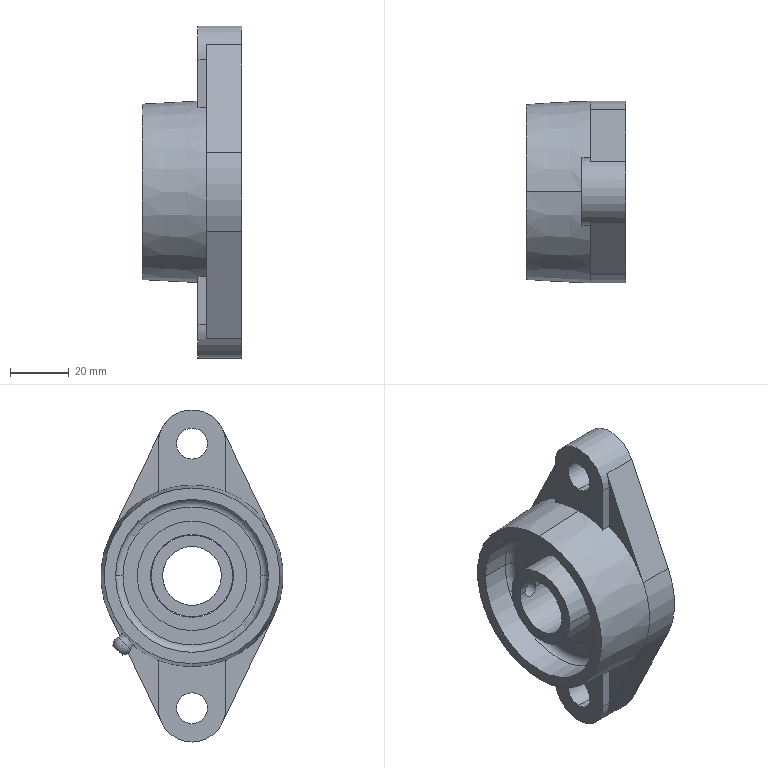Component | SolidWorks | BearingWithRhombicSeatUCFLU204-1 | 1 solid | 91 faces | volume 69605 mm3 | cylinder 40 | plane 33 | sphere 10 | torus 6 | cone 2 | commonest cylinder face diameters 37.28 x6 23 x6 6 x6 28.23 x4 52 x4 10.5 x4 5.35 x2 27.83 x2